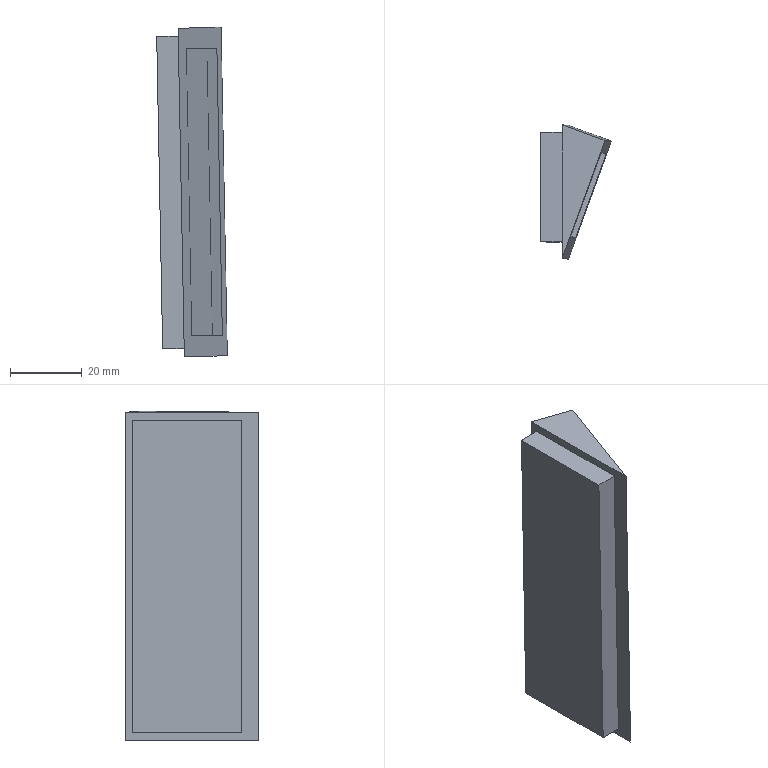Component | SolidWorks | 93X35EmbeddedHandleSlot87X30.5-16 | 1 solid | 15 faces | box 19.67 x 37.25 x 91.71 mm | volume 30319 mm3 | plane 15 | material A3 Steel
STEP:
#1=COLOUR_RGB('',0.7922,0.8196,0.9333);
#2=FILL_AREA_STYLE_COLOUR('',#1);
#3=FILL_AREA_STYLE('',(#2));
#4=SURFACE_STYLE_FILL_AREA(#3);
#5=SURFACE_SIDE_STYLE('',(#4));
#6=SURFACE_STYLE_USAGE(.BOTH.,#5);
#7=PRESENTATION_STYLE_ASSIGNMENT((#6));
#8=CARTESIAN_POINT('',(39.387,-70.188,66.165));
#9=VERTEX_POINT('',#8);
#10=CARTESIAN_POINT('',(39.387,-71.389,66.165));
#11=VERTEX_POINT('',#10);
#12=CARTESIAN_POINT('',(39.387,-70.188,66.165));
#13=DIRECTION('',(0.,-1.,0.));
#14=VECTOR('',#13,39.37);
#15=LINE('',#12,#14);
#16=EDGE_CURVE('',#9,#11,#15,.T.);
#17=ORIENTED_EDGE('',*,*,#16,.T.);
#18=CARTESIAN_POINT('',(39.151,-71.389,66.161));
#19=VERTEX_POINT('',#18);
#20=CARTESIAN_POINT('',(39.151,-71.389,66.161));
#21=DIRECTION('',(0.9998,0.,0.01904));
#22=VECTOR('',#21,39.37);
#23=LINE('',#20,#22);
#24=EDGE_CURVE('',#19,#11,#23,.T.);
#25=ORIENTED_EDGE('',*,*,#24,.F.);
#26=CARTESIAN_POINT('',(39.151,-70.188,66.161));
#27=VERTEX_POINT('',#26);
#28=CARTESIAN_POINT('',(39.151,-70.188,66.161));
#29=DIRECTION('',(0.,-1.,0.));
#30=VECTOR('',#29,39.37);
#31=LINE('',#28,#30);
#32=EDGE_CURVE('',#27,#19,#31,.T.);
#33=ORIENTED_EDGE('',*,*,#32,.F.);
#34=CARTESIAN_POINT('',(39.151,-70.188,66.161));
#35=DIRECTION('',(0.9998,0.,0.01904));
#36=VECTOR('',#35,39.37);
#37=LINE('',#34,#36);
#38=EDGE_CURVE('',#27,#9,#37,.T.);
#39=ORIENTED_EDGE('',*,*,#38,.T.);
#40=EDGE_LOOP('',(#17,#25,#33,#39));
#41=FACE_OUTER_BOUND('',#40,.T.);
#42=CARTESIAN_POINT('',(39.151,-70.188,66.161));
#43=DIRECTION('',(-0.01904,0.,0.9998));
#44=DIRECTION('',(-0.9998,-0.,-0.01904));
#45=AXIS2_PLACEMENT_3D('',#42,#43,#44);
#46=PLANE('',#45);
#47=ADVANCED_FACE('',(#41),#46,.F.);
#48=CARTESIAN_POINT('',(39.322,-71.389,69.59));
#49=VERTEX_POINT('',#48);
#50=CARTESIAN_POINT('',(39.322,-71.389,69.59));
#51=DIRECTION('',(-0.01904,0.,0.9998));
#52=VECTOR('',#51,39.37);
#53=LINE('',#50,#52);
#54=EDGE_CURVE('',#11,#49,#53,.T.);
#55=ORIENTED_EDGE('',*,*,#54,.T.);
#56=CARTESIAN_POINT('',(39.085,-71.389,69.585));
#57=VERTEX_POINT('',#56);
#58=CARTESIAN_POINT('',(39.085,-71.389,69.585));
#59=DIRECTION('',(0.9998,0.,0.01904));
#60=VECTOR('',#59,39.37);
#61=LINE('',#58,#60);
#62=EDGE_CURVE('',#57,#49,#61,.T.);
#63=ORIENTED_EDGE('',*,*,#62,.F.);
#64=CARTESIAN_POINT('',(39.085,-71.389,69.585));
#65=DIRECTION('',(-0.01904,0.,0.9998));
#66=VECTOR('',#65,39.37);
#67=LINE('',#64,#66);
#68=EDGE_CURVE('',#19,#57,#67,.T.);
#69=ORIENTED_EDGE('',*,*,#68,.F.);
#70=ORIENTED_EDGE('',*,*,#24,.T.);
#71=EDGE_LOOP('',(#55,#63,#69,#70));
#72=FACE_OUTER_BOUND('',#71,.T.);
#73=CARTESIAN_POINT('',(39.085,-71.389,69.585));
#74=DIRECTION('',(-0.,1.,-0.));
#75=DIRECTION('',(0.9998,0.,0.01904));
#76=AXIS2_PLACEMENT_3D('',#73,#74,#75);
#77=PLANE('',#76);
#78=ADVANCED_FACE('',(#72),#77,.F.);
#79=CARTESIAN_POINT('',(39.322,-70.188,69.59));
#80=VERTEX_POINT('',#79);
#81=CARTESIAN_POINT('',(39.322,-70.188,69.59));
#82=DIRECTION('',(-0.,1.,-0.));
#83=VECTOR('',#82,39.37);
#84=LINE('',#81,#83);
#85=EDGE_CURVE('',#49,#80,#84,.T.);
#86=ORIENTED_EDGE('',*,*,#85,.T.);
#87=CARTESIAN_POINT('',(39.085,-70.188,69.585));
#88=VERTEX_POINT('',#87);
#89=CARTESIAN_POINT('',(39.085,-70.188,69.585));
#90=DIRECTION('',(0.9998,0.,0.01904));
#91=VECTOR('',#90,39.37);
#92=LINE('',#89,#91);
#93=EDGE_CURVE('',#88,#80,#92,.T.);
#94=ORIENTED_EDGE('',*,*,#93,.F.);
#95=CARTESIAN_POINT('',(39.085,-70.188,69.585));
#96=DIRECTION('',(-0.,1.,-0.));
#97=VECTOR('',#96,39.37);
#98=LINE('',#95,#97);
#99=EDGE_CURVE('',#57,#88,#98,.T.);
#100=ORIENTED_EDGE('',*,*,#99,.F.);
#101=ORIENTED_EDGE('',*,*,#62,.T.);
#102=EDGE_LOOP('',(#86,#94,#100,#101));
#103=FACE_OUTER_BOUND('',#102,.T.);
#104=CARTESIAN_POINT('',(39.085,-70.188,69.585));
#105=DIRECTION('',(0.01904,-0.,-0.9998));
#106=DIRECTION('',(0.9998,0.,0.01904));
#107=AXIS2_PLACEMENT_3D('',#104,#105,#106);
#108=PLANE('',#107);
#109=ADVANCED_FACE('',(#103),#108,.F.);
#110=CARTESIAN_POINT('',(39.322,-70.188,69.59));
#111=DIRECTION('',(0.01904,-0.,-0.9998));
#112=VECTOR('',#111,39.37);
#113=LINE('',#110,#112);
#114=EDGE_CURVE('',#80,#9,#113,.T.);
#115=ORIENTED_EDGE('',*,*,#114,.T.);
#116=ORIENTED_EDGE('',*,*,#38,.F.);
#117=CARTESIAN_POINT('',(39.085,-70.188,69.585));
#118=DIRECTION('',(0.01904,-0.,-0.9998));
#119=VECTOR('',#118,39.37);
#120=LINE('',#117,#119);
#121=EDGE_CURVE('',#88,#27,#120,.T.);
#122=ORIENTED_EDGE('',*,*,#121,.F.);
#123=ORIENTED_EDGE('',*,*,#93,.T.);
#124=EDGE_LOOP('',(#115,#116,#122,#123));
#125=FACE_OUTER_BOUND('',#124,.T.);
#126=CARTESIAN_POINT('',(39.085,-70.188,69.585));
#127=DIRECTION('',(0.,-1.,0.));
#128=DIRECTION('',(-0.9998,-0.,-0.01904));
#129=AXIS2_PLACEMENT_3D('',#126,#127,#128);
#130=PLANE('',#129);
#131=ADVANCED_FACE('',(#125),#130,.F.);
#132=ORIENTED_EDGE('',*,*,#32,.T.);
#133=ORIENTED_EDGE('',*,*,#68,.T.);
#134=ORIENTED_EDGE('',*,*,#99,.T.);
#135=ORIENTED_EDGE('',*,*,#121,.T.);
#136=EDGE_LOOP('',(#132,#133,#134,#135));
#137=FACE_OUTER_BOUND('',#136,.T.);
#138=CARTESIAN_POINT('',(39.118,-70.788,67.873));
#139=DIRECTION('',(0.9998,0.,0.01904));
#140=DIRECTION('',(-0.01904,0.,0.9998));
#141=AXIS2_PLACEMENT_3D('',#138,#139,#140);
#142=PLANE('',#141);
#143=ADVANCED_FACE('',(#137),#142,.F.);
#144=CARTESIAN_POINT('',(39.32,-70.109,69.678));
#145=VERTEX_POINT('',#144);
#146=CARTESIAN_POINT('',(39.32,-71.576,69.678));
#147=VERTEX_POINT('',#146);
#148=CARTESIAN_POINT('',(39.32,-70.109,69.678));
#149=DIRECTION('',(0.,-1.,0.));
#150=VECTOR('',#149,39.37);
#151=LINE('',#148,#150);
#152=EDGE_CURVE('',#145,#147,#151,.T.);
#153=ORIENTED_EDGE('',*,*,#152,.F.);
#154=CARTESIAN_POINT('',(39.388,-70.109,66.077));
#155=VERTEX_POINT('',#154);
#156=CARTESIAN_POINT('',(39.388,-70.109,66.077));
#157=DIRECTION('',(-0.01904,0.,0.9998));
#158=VECTOR('',#157,39.37);
#159=LINE('',#156,#158);
#160=EDGE_CURVE('',#155,#145,#159,.T.);
#161=ORIENTED_EDGE('',*,*,#160,.F.);
#162=CARTESIAN_POINT('',(39.388,-71.576,66.077));
#163=VERTEX_POINT('',#162);
#164=CARTESIAN_POINT('',(39.388,-71.576,66.077));
#165=DIRECTION('',(-0.,1.,-0.));
#166=VECTOR('',#165,39.37);
#167=LINE('',#164,#166);
#168=EDGE_CURVE('',#163,#155,#167,.T.);
#169=ORIENTED_EDGE('',*,*,#168,.F.);
#170=CARTESIAN_POINT('',(39.388,-71.576,66.077));
#171=DIRECTION('',(-0.01904,0.,0.9998));
#172=VECTOR('',#171,39.37);
#173=LINE('',#170,#172);
#174=EDGE_CURVE('',#163,#147,#173,.T.);
#175=ORIENTED_EDGE('',*,*,#174,.T.);
#176=EDGE_LOOP('',(#153,#161,#169,#175));
#177=FACE_OUTER_BOUND('',#176,.T.);
#178=ORIENTED_EDGE('',*,*,#16,.F.);
#179=ORIENTED_EDGE('',*,*,#114,.F.);
#180=ORIENTED_EDGE('',*,*,#85,.F.);
#181=ORIENTED_EDGE('',*,*,#54,.F.);
#182=EDGE_LOOP('',(#178,#179,#180,#181));
#183=FACE_BOUND('',#182,.T.);
#184=CARTESIAN_POINT('',(39.388,-70.109,66.077));
#185=DIRECTION('',(-0.9998,-0.,-0.01904));
#186=DIRECTION('',(-0.,1.,-0.));
#187=AXIS2_PLACEMENT_3D('',#184,#185,#186);
#188=PLANE('',#187);
#189=ADVANCED_FACE('',(#177,#183),#188,.T.);
#190=CARTESIAN_POINT('',(39.791,-70.281,69.687));
#191=VERTEX_POINT('',#190);
#192=CARTESIAN_POINT('',(39.791,-70.281,69.687));
#193=DIRECTION('',(-0.9395,0.342,-0.0179));
#194=VECTOR('',#193,39.37);
#195=LINE('',#192,#194);
#196=EDGE_CURVE('',#191,#145,#195,.T.);
#197=ORIENTED_EDGE('',*,*,#196,.F.);
#198=CARTESIAN_POINT('',(39.86,-70.281,66.086));
#199=VERTEX_POINT('',#198);
#200=CARTESIAN_POINT('',(39.86,-70.281,66.086));
#201=DIRECTION('',(-0.01904,0.,0.9998));
#202=VECTOR('',#201,39.37);
#203=LINE('',#200,#202);
#204=EDGE_CURVE('',#199,#191,#203,.T.);
#205=ORIENTED_EDGE('',*,*,#204,.F.);
#206=CARTESIAN_POINT('',(39.86,-70.281,66.086));
#207=DIRECTION('',(-0.9395,0.342,-0.0179));
#208=VECTOR('',#207,39.37);
#209=LINE('',#206,#208);
#210=EDGE_CURVE('',#199,#155,#209,.T.);
#211=ORIENTED_EDGE('',*,*,#210,.T.);
#212=ORIENTED_EDGE('',*,*,#160,.T.);
#213=EDGE_LOOP('',(#197,#205,#211,#212));
#214=FACE_OUTER_BOUND('',#213,.T.);
#215=CARTESIAN_POINT('',(39.86,-70.281,66.086));
#216=DIRECTION('',(0.342,0.9397,0.006514));
#217=DIRECTION('',(0.9395,-0.342,0.0179));
#218=AXIS2_PLACEMENT_3D('',#215,#216,#217);
#219=PLANE('',#218);
#220=ADVANCED_FACE('',(#214),#219,.T.);
#221=CARTESIAN_POINT('',(39.745,-70.418,69.46));
#222=VERTEX_POINT('',#221);
#223=CARTESIAN_POINT('',(39.409,-71.343,69.454));
#224=VERTEX_POINT('',#223);
#225=CARTESIAN_POINT('',(39.745,-70.418,69.46));
#226=DIRECTION('',(-0.342,-0.9397,-0.006514));
#227=VECTOR('',#226,39.37);
#228=LINE('',#225,#227);
#229=EDGE_CURVE('',#222,#224,#228,.T.);
#230=ORIENTED_EDGE('',*,*,#229,.F.);
#231=CARTESIAN_POINT('',(39.805,-70.418,66.311));
#232=VERTEX_POINT('',#231);
#233=CARTESIAN_POINT('',(39.805,-70.418,66.311));
#234=DIRECTION('',(-0.01904,0.,0.9998));
#235=VECTOR('',#234,39.37);
#236=LINE('',#233,#235);
#237=EDGE_CURVE('',#232,#222,#236,.T.);
#238=ORIENTED_EDGE('',*,*,#237,.F.);
#239=CARTESIAN_POINT('',(39.469,-71.343,66.305));
#240=VERTEX_POINT('',#239);
#241=CARTESIAN_POINT('',(39.805,-70.418,66.311));
#242=DIRECTION('',(0.342,0.9397,0.006514));
#243=VECTOR('',#242,39.37);
#244=LINE('',#241,#243);
#245=EDGE_CURVE('',#240,#232,#244,.T.);
#246=ORIENTED_EDGE('',*,*,#245,.F.);
#247=CARTESIAN_POINT('',(39.469,-71.343,66.305));
#248=DIRECTION('',(0.01904,-0.,-0.9998));
#249=VECTOR('',#248,39.37);
#250=LINE('',#247,#249);
#251=EDGE_CURVE('',#224,#240,#250,.T.);
#252=ORIENTED_EDGE('',*,*,#251,.F.);
#253=EDGE_LOOP('',(#230,#238,#246,#252));
#254=FACE_BOUND('',#253,.T.);
#255=CARTESIAN_POINT('',(39.32,-71.576,69.678));
#256=DIRECTION('',(0.342,0.9397,0.006514));
#257=VECTOR('',#256,39.37);
#258=LINE('',#255,#257);
#259=EDGE_CURVE('',#147,#191,#258,.T.);
#260=ORIENTED_EDGE('',*,*,#259,.F.);
#261=ORIENTED_EDGE('',*,*,#174,.F.);
#262=CARTESIAN_POINT('',(39.388,-71.576,66.077));
#263=DIRECTION('',(0.342,0.9397,0.006514));
#264=VECTOR('',#263,39.37);
#265=LINE('',#262,#264);
#266=EDGE_CURVE('',#163,#199,#265,.T.);
#267=ORIENTED_EDGE('',*,*,#266,.T.);
#268=ORIENTED_EDGE('',*,*,#204,.T.);
#269=EDGE_LOOP('',(#260,#261,#267,#268));
#270=FACE_OUTER_BOUND('',#269,.T.);
#271=CARTESIAN_POINT('',(39.388,-71.576,66.077));
#272=DIRECTION('',(0.9395,-0.342,0.0179));
#273=DIRECTION('',(-0.342,-0.9397,-0.006514));
#274=AXIS2_PLACEMENT_3D('',#271,#272,#273);
#275=PLANE('',#274);
#276=ADVANCED_FACE('',(#254,#270),#275,.T.);
#277=ORIENTED_EDGE('',*,*,#168,.T.);
#278=ORIENTED_EDGE('',*,*,#210,.F.);
#279=ORIENTED_EDGE('',*,*,#266,.F.);
#280=EDGE_LOOP('',(#277,#278,#279));
#281=FACE_OUTER_BOUND('',#280,.T.);
#282=CARTESIAN_POINT('',(39.388,-70.788,66.077));
#283=DIRECTION('',(-0.01904,0.,0.9998));
#284=DIRECTION('',(-0.9998,-0.,-0.01904));
#285=AXIS2_PLACEMENT_3D('',#282,#283,#284);
#286=PLANE('',#285);
#287=ADVANCED_FACE('',(#281),#286,.F.);
#288=ORIENTED_EDGE('',*,*,#152,.T.);
#289=ORIENTED_EDGE('',*,*,#259,.T.);
#290=ORIENTED_EDGE('',*,*,#196,.T.);
#291=EDGE_LOOP('',(#288,#289,#290));
#292=FACE_OUTER_BOUND('',#291,.T.);
#293=CARTESIAN_POINT('',(39.32,-70.788,69.678));
#294=DIRECTION('',(-0.01904,0.,0.9998));
#295=DIRECTION('',(-0.9998,-0.,-0.01904));
#296=AXIS2_PLACEMENT_3D('',#293,#294,#295);
#297=PLANE('',#296);
#298=ADVANCED_FACE('',(#292),#297,.T.);
#299=ORIENTED_EDGE('',*,*,#229,.T.);
#300=CARTESIAN_POINT('',(39.298,-71.302,69.452));
#301=VERTEX_POINT('',#300);
#302=CARTESIAN_POINT('',(39.298,-71.302,69.452));
#303=DIRECTION('',(0.9395,-0.342,0.0179));
#304=VECTOR('',#303,39.37);
#305=LINE('',#302,#304);
#306=EDGE_CURVE('',#301,#224,#305,.T.);
#307=ORIENTED_EDGE('',*,*,#306,.F.);
#308=CARTESIAN_POINT('',(39.634,-70.378,69.458));
#309=VERTEX_POINT('',#308);
#310=CARTESIAN_POINT('',(39.634,-70.378,69.458));
#311=DIRECTION('',(-0.342,-0.9397,-0.006514));
#312=VECTOR('',#311,39.37);
#313=LINE('',#310,#312);
#314=EDGE_CURVE('',#309,#301,#313,.T.);
#315=ORIENTED_EDGE('',*,*,#314,.F.);
#316=CARTESIAN_POINT('',(39.634,-70.378,69.458));
#317=DIRECTION('',(0.9395,-0.342,0.0179));
#318=VECTOR('',#317,39.37);
#319=LINE('',#316,#318);
#320=EDGE_CURVE('',#309,#222,#319,.T.);
#321=ORIENTED_EDGE('',*,*,#320,.T.);
#322=EDGE_LOOP('',(#299,#307,#315,#321));
#323=FACE_OUTER_BOUND('',#322,.T.);
#324=CARTESIAN_POINT('',(39.634,-70.378,69.458));
#325=DIRECTION('',(-0.01904,0.,0.9998));
#326=DIRECTION('',(-0.9998,-0.,-0.01904));
#327=AXIS2_PLACEMENT_3D('',#324,#325,#326);
#328=PLANE('',#327);
#329=ADVANCED_FACE('',(#323),#328,.F.);
#330=ORIENTED_EDGE('',*,*,#237,.T.);
#331=ORIENTED_EDGE('',*,*,#320,.F.);
#332=CARTESIAN_POINT('',(39.694,-70.378,66.309));
#333=VERTEX_POINT('',#332);
#334=CARTESIAN_POINT('',(39.694,-70.378,66.309));
#335=DIRECTION('',(-0.01904,0.,0.9998));
#336=VECTOR('',#335,39.37);
#337=LINE('',#334,#336);
#338=EDGE_CURVE('',#333,#309,#337,.T.);
#339=ORIENTED_EDGE('',*,*,#338,.F.);
#340=CARTESIAN_POINT('',(39.694,-70.378,66.309));
#341=DIRECTION('',(0.9395,-0.342,0.0179));
#342=VECTOR('',#341,39.37);
#343=LINE('',#340,#342);
#344=EDGE_CURVE('',#333,#232,#343,.T.);
#345=ORIENTED_EDGE('',*,*,#344,.T.);
#346=EDGE_LOOP('',(#330,#331,#339,#345));
#347=FACE_OUTER_BOUND('',#346,.T.);
#348=CARTESIAN_POINT('',(39.694,-70.378,66.309));
#349=DIRECTION('',(0.342,0.9397,0.006514));
#350=DIRECTION('',(0.9395,-0.342,0.0179));
#351=AXIS2_PLACEMENT_3D('',#348,#349,#350);
#352=PLANE('',#351);
#353=ADVANCED_FACE('',(#347),#352,.F.);
#354=ORIENTED_EDGE('',*,*,#245,.T.);
#355=ORIENTED_EDGE('',*,*,#344,.F.);
#356=CARTESIAN_POINT('',(39.358,-71.302,66.303));
#357=VERTEX_POINT('',#356);
#358=CARTESIAN_POINT('',(39.694,-70.378,66.309));
#359=DIRECTION('',(0.342,0.9397,0.006514));
#360=VECTOR('',#359,39.37);
#361=LINE('',#358,#360);
#362=EDGE_CURVE('',#357,#333,#361,.T.);
#363=ORIENTED_EDGE('',*,*,#362,.F.);
#364=CARTESIAN_POINT('',(39.358,-71.302,66.303));
#365=DIRECTION('',(0.9395,-0.342,0.0179));
#366=VECTOR('',#365,39.37);
#367=LINE('',#364,#366);
#368=EDGE_CURVE('',#357,#240,#367,.T.);
#369=ORIENTED_EDGE('',*,*,#368,.T.);
#370=EDGE_LOOP('',(#354,#355,#363,#369));
#371=FACE_OUTER_BOUND('',#370,.T.);
#372=CARTESIAN_POINT('',(39.694,-70.378,66.309));
#373=DIRECTION('',(0.01904,-0.,-0.9998));
#374=DIRECTION('',(0.9998,0.,0.01904));
#375=AXIS2_PLACEMENT_3D('',#372,#373,#374);
#376=PLANE('',#375);
#377=ADVANCED_FACE('',(#371),#376,.F.);
#378=ORIENTED_EDGE('',*,*,#251,.T.);
#379=ORIENTED_EDGE('',*,*,#368,.F.);
#380=CARTESIAN_POINT('',(39.358,-71.302,66.303));
#381=DIRECTION('',(0.01904,-0.,-0.9998));
#382=VECTOR('',#381,39.37);
#383=LINE('',#380,#382);
#384=EDGE_CURVE('',#301,#357,#383,.T.);
#385=ORIENTED_EDGE('',*,*,#384,.F.);
#386=ORIENTED_EDGE('',*,*,#306,.T.);
#387=EDGE_LOOP('',(#378,#379,#385,#386));
#388=FACE_OUTER_BOUND('',#387,.T.);
#389=CARTESIAN_POINT('',(39.358,-71.302,66.303));
#390=DIRECTION('',(-0.342,-0.9397,-0.006514));
#391=DIRECTION('',(-0.9395,0.342,-0.0179));
#392=AXIS2_PLACEMENT_3D('',#389,#390,#391);
#393=PLANE('',#392);
#394=ADVANCED_FACE('',(#388),#393,.F.);
#395=ORIENTED_EDGE('',*,*,#314,.T.);
#396=ORIENTED_EDGE('',*,*,#384,.T.);
#397=ORIENTED_EDGE('',*,*,#362,.T.);
#398=ORIENTED_EDGE('',*,*,#338,.T.);
#399=EDGE_LOOP('',(#395,#396,#397,#398));
#400=FACE_OUTER_BOUND('',#399,.T.);
#401=CARTESIAN_POINT('',(39.496,-70.84,67.88));
#402=DIRECTION('',(-0.9395,0.342,-0.0179));
#403=DIRECTION('',(0.342,0.9397,0.006514));
#404=AXIS2_PLACEMENT_3D('',#401,#402,#403);
#405=PLANE('',#404);
#406=ADVANCED_FACE('',(#400),#405,.F.);
#407=CLOSED_SHELL('',(#47,#78,#109,#131,#143,#189,#220,#276,#287,#298,#329,#353,#377,#394,#406));
#408=MANIFOLD_SOLID_BREP('',#407);
#409=STYLED_ITEM('',(#7),#408);
#410=PRESENTATION_LAYER_ASSIGNMENT('','',(#409));
#411=CARTESIAN_POINT('',(0.,0.,0.));
#412=DIRECTION('',(0.,0.,1.));
#413=DIRECTION('',(1.,0.,0.));
#414=AXIS2_PLACEMENT_3D('',#411,#412,#413);
#415=(LENGTH_UNIT()NAMED_UNIT(*)SI_UNIT($,.METRE.));
#416=LENGTH_MEASURE_WITH_UNIT(LENGTH_MEASURE(0.0254),#415);
#417=DIMENSIONAL_EXPONENTS(1.,0.,0.,0.,0.,0.,0.);
#418=(CONVERSION_BASED_UNIT('',#416)LENGTH_UNIT()NAMED_UNIT(#417));
#419=UNCERTAINTY_MEASURE_WITH_UNIT(LENGTH_MEASURE(0.00001),#418,'','');
#420=(NAMED_UNIT(*)PLANE_ANGLE_UNIT()SI_UNIT($,.RADIAN.));
#421=(NAMED_UNIT(*)SI_UNIT($,.STERADIAN.)SOLID_ANGLE_UNIT());
#422=(GEOMETRIC_REPRESENTATION_CONTEXT(3)GLOBAL_UNCERTAINTY_ASSIGNED_CONTEXT((#419))GLOBAL_UNIT_ASSIGNED_CONTEXT((#418,#420,#421))REPRESENTATION_CONTEXT('',''));
#423=ADVANCED_BREP_SHAPE_REPRESENTATION('',(#408,#414),#422);
#424=(LENGTH_UNIT()NAMED_UNIT(*)SI_UNIT($,.METRE.));
#425=LENGTH_MEASURE_WITH_UNIT(LENGTH_MEASURE(0.0254),#424);
#426=DIMENSIONAL_EXPONENTS(1.,0.,0.,0.,0.,0.,0.);
#427=(CONVERSION_BASED_UNIT('',#425)LENGTH_UNIT()NAMED_UNIT(#426));
#428=UNCERTAINTY_MEASURE_WITH_UNIT(LENGTH_MEASURE(0.00001),#427,'','');
#429=(NAMED_UNIT(*)PLANE_ANGLE_UNIT()SI_UNIT($,.RADIAN.));
#430=(NAMED_UNIT(*)SI_UNIT($,.STERADIAN.)SOLID_ANGLE_UNIT());
#431=(GEOMETRIC_REPRESENTATION_CONTEXT(3)GLOBAL_UNCERTAINTY_ASSIGNED_CONTEXT((#428))GLOBAL_UNIT_ASSIGNED_CONTEXT((#427,#429,#430))REPRESENTATION_CONTEXT('',''));
#432=MECHANICAL_DESIGN_GEOMETRIC_PRESENTATION_REPRESENTATION('',(#409),#431);